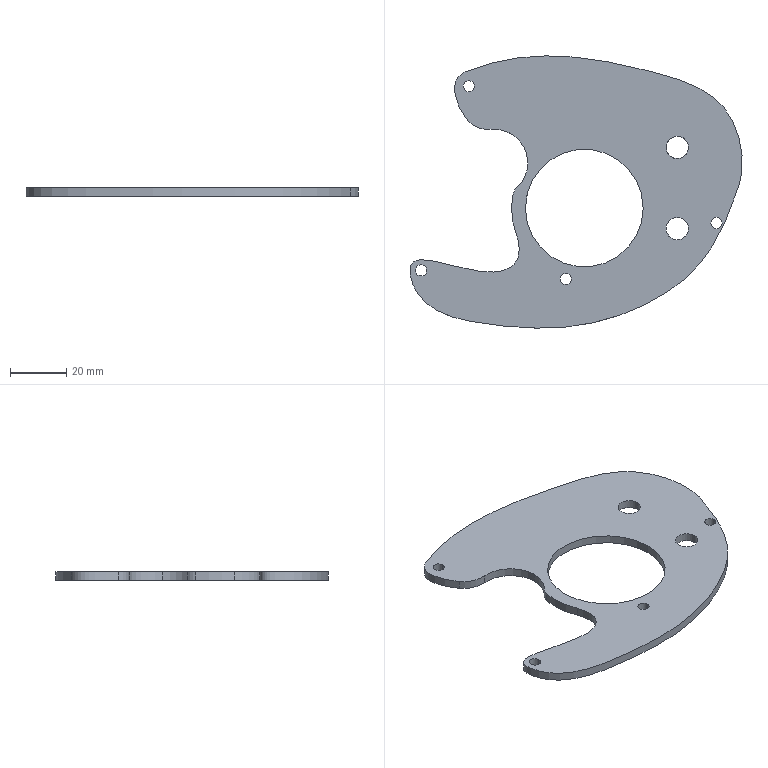Component | SolidWorks | Sub-plate-3 | 1 solid | 24 faces | volume 17941 mm3 | cylinder 19 | spline 3 | plane 2 | commonest cylinder face diameters 4 x8 8 x4 24 x2 42 x2 20 x1 10 x1 52 x1